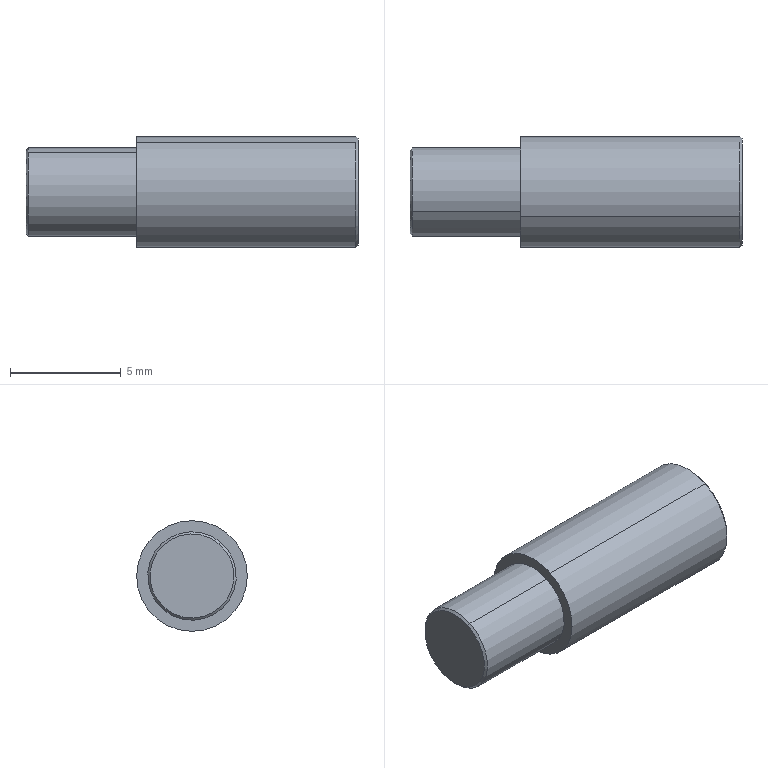Component | SolidWorks | F01AE00111-A2000-21TopEdgeAssembly-1_F01AE00111-A2000-19TopEdgeRollerAssembly-1_F01AE00111-A2008-1 | 1 solid | 11 faces | box 15 x 5 x 5 mm | volume 259 mm3 | cone 4 | cylinder 4 | plane 3 | commonest cylinder face diameters 5 x2 4 x2 | material AISI 304
build123d program:
from build123d import *

# Parameters (mm, degrees)
CHAMFER1_SIZE = 0.1


with BuildPart() as part:
    # Sketch1 → Revolve1 (revolve)
    with BuildSketch(Plane.XY, mode=Mode.PRIVATE) as revolve1_sk:
        Polygon((0, 15), (2, 15), (2, 10), (2.5, 10), (2.5, 0), (0, 0), align=None)
    revolve(revolve1_sk.sketch.rotate(Axis((0, 0, 0), (0, 1, 0)), 90), axis=Axis((0, 0, 0), (0, 1, 0)))

    # Chamfer1
    chamfer1_edges = [part.edges().sort_by_distance(p)[0] for p in [
        (0, 0, 2.5),
        (0, 15, 2),
    ]]
    chamfer(chamfer1_edges, length=CHAMFER1_SIZE)


solid = part.part

# Placed as in the assembly
solid = solid.moved(Location((-133.852, 75.398, -381.975), (0, 0, 90)))
STEP:
#1=COLOUR_RGB('',0.7922,0.8196,0.9333);
#2=FILL_AREA_STYLE_COLOUR('',#1);
#3=FILL_AREA_STYLE('',(#2));
#4=SURFACE_STYLE_FILL_AREA(#3);
#5=SURFACE_SIDE_STYLE('',(#4));
#6=SURFACE_STYLE_USAGE(.BOTH.,#5);
#7=PRESENTATION_STYLE_ASSIGNMENT((#6));
#8=CARTESIAN_POINT('',(-5.86,2.936,-14.971));
#9=VERTEX_POINT('',#8);
#10=CARTESIAN_POINT('',(-5.86,3.001,-15.106));
#11=VERTEX_POINT('',#10);
#12=CARTESIAN_POINT('',(-5.86,2.968,-15.038));
#13=DIRECTION('',(-1.,-0.,-0.));
#14=DIRECTION('',(0.,-0.4399,0.898));
#15=AXIS2_PLACEMENT_3D('',#12,#13,#14);
#16=CIRCLE('',#15,0.0748);
#17=EDGE_CURVE('',#9,#11,#16,.T.);
#18=ORIENTED_EDGE('',*,*,#17,.F.);
#19=CARTESIAN_POINT('',(-5.856,2.934,-14.968));
#20=VERTEX_POINT('',#19);
#21=CARTESIAN_POINT('',(-5.856,2.934,-14.968));
#22=DIRECTION('',(0.7071,-0.3111,0.635));
#23=VECTOR('',#22,39.37);
#24=LINE('',#21,#23);
#25=EDGE_CURVE('',#9,#20,#24,.T.);
#26=ORIENTED_EDGE('',*,*,#25,.T.);
#27=CARTESIAN_POINT('',(-5.856,3.003,-15.109));
#28=VERTEX_POINT('',#27);
#29=CARTESIAN_POINT('',(-5.856,2.968,-15.038));
#30=DIRECTION('',(1.,0.,0.));
#31=DIRECTION('',(0.,-0.4399,0.898));
#32=AXIS2_PLACEMENT_3D('',#29,#30,#31);
#33=CIRCLE('',#32,0.07874);
#34=EDGE_CURVE('',#28,#20,#33,.T.);
#35=ORIENTED_EDGE('',*,*,#34,.F.);
#36=CARTESIAN_POINT('',(-5.856,3.003,-15.109));
#37=DIRECTION('',(0.7071,0.3111,-0.635));
#38=VECTOR('',#37,39.37);
#39=LINE('',#36,#38);
#40=EDGE_CURVE('',#11,#28,#39,.T.);
#41=ORIENTED_EDGE('',*,*,#40,.F.);
#42=EDGE_LOOP('',(#18,#26,#35,#41));
#43=FACE_OUTER_BOUND('',#42,.T.);
#44=CARTESIAN_POINT('',(-5.856,2.968,-15.038));
#45=DIRECTION('',(1.,0.,0.));
#46=DIRECTION('',(0.,0.4399,-0.898));
#47=AXIS2_PLACEMENT_3D('',#44,#45,#46);
#48=CONICAL_SURFACE('',#47,0.07874,0.7854);
#49=ADVANCED_FACE('',(#43),#48,.T.);
#50=CARTESIAN_POINT('',(-5.27,3.01,-15.123));
#51=VERTEX_POINT('',#50);
#52=CARTESIAN_POINT('',(-5.27,2.927,-14.954));
#53=VERTEX_POINT('',#52);
#54=CARTESIAN_POINT('',(-5.27,2.968,-15.038));
#55=DIRECTION('',(1.,0.,0.));
#56=DIRECTION('',(0.,0.4399,-0.898));
#57=AXIS2_PLACEMENT_3D('',#54,#55,#56);
#58=CIRCLE('',#57,0.09449);
#59=EDGE_CURVE('',#51,#53,#58,.T.);
#60=ORIENTED_EDGE('',*,*,#59,.F.);
#61=CARTESIAN_POINT('',(-5.274,3.012,-15.127));
#62=VERTEX_POINT('',#61);
#63=CARTESIAN_POINT('',(-5.27,3.01,-15.123));
#64=DIRECTION('',(-0.7071,0.3111,-0.635));
#65=VECTOR('',#64,39.37);
#66=LINE('',#63,#65);
#67=EDGE_CURVE('',#51,#62,#66,.T.);
#68=ORIENTED_EDGE('',*,*,#67,.T.);
#69=CARTESIAN_POINT('',(-5.274,2.925,-14.95));
#70=VERTEX_POINT('',#69);
#71=CARTESIAN_POINT('',(-5.274,2.968,-15.038));
#72=DIRECTION('',(-1.,-0.,-0.));
#73=DIRECTION('',(0.,0.4399,-0.898));
#74=AXIS2_PLACEMENT_3D('',#71,#72,#73);
#75=CIRCLE('',#74,0.09843);
#76=EDGE_CURVE('',#70,#62,#75,.T.);
#77=ORIENTED_EDGE('',*,*,#76,.F.);
#78=CARTESIAN_POINT('',(-5.27,2.927,-14.954));
#79=DIRECTION('',(-0.7071,-0.3111,0.635));
#80=VECTOR('',#79,39.37);
#81=LINE('',#78,#80);
#82=EDGE_CURVE('',#53,#70,#81,.T.);
#83=ORIENTED_EDGE('',*,*,#82,.F.);
#84=EDGE_LOOP('',(#60,#68,#77,#83));
#85=FACE_OUTER_BOUND('',#84,.T.);
#86=CARTESIAN_POINT('',(-5.27,2.968,-15.038));
#87=DIRECTION('',(-1.,-0.,-0.));
#88=DIRECTION('',(0.,-0.4399,0.898));
#89=AXIS2_PLACEMENT_3D('',#86,#87,#88);
#90=CONICAL_SURFACE('',#89,0.09449,0.7854);
#91=ADVANCED_FACE('',(#85),#90,.T.);
#92=CARTESIAN_POINT('',(-5.663,3.012,-15.127));
#93=VERTEX_POINT('',#92);
#94=CARTESIAN_POINT('',(-5.663,2.925,-14.95));
#95=VERTEX_POINT('',#94);
#96=CARTESIAN_POINT('',(-5.663,2.968,-15.038));
#97=DIRECTION('',(1.,0.,0.));
#98=DIRECTION('',(0.,0.4399,-0.898));
#99=AXIS2_PLACEMENT_3D('',#96,#97,#98);
#100=CIRCLE('',#99,0.09843);
#101=EDGE_CURVE('',#93,#95,#100,.T.);
#102=ORIENTED_EDGE('',*,*,#101,.T.);
#103=CARTESIAN_POINT('',(-5.27,2.925,-14.95));
#104=DIRECTION('',(1.,0.,0.));
#105=VECTOR('',#104,39.37);
#106=LINE('',#103,#105);
#107=EDGE_CURVE('',#95,#70,#106,.T.);
#108=ORIENTED_EDGE('',*,*,#107,.T.);
#109=ORIENTED_EDGE('',*,*,#76,.T.);
#110=CARTESIAN_POINT('',(-5.27,3.012,-15.127));
#111=DIRECTION('',(1.,0.,0.));
#112=VECTOR('',#111,39.37);
#113=LINE('',#110,#112);
#114=EDGE_CURVE('',#93,#62,#113,.T.);
#115=ORIENTED_EDGE('',*,*,#114,.F.);
#116=EDGE_LOOP('',(#102,#108,#109,#115));
#117=FACE_OUTER_BOUND('',#116,.T.);
#118=CARTESIAN_POINT('',(-5.27,2.968,-15.038));
#119=DIRECTION('',(1.,0.,0.));
#120=DIRECTION('',(0.,0.4399,-0.898));
#121=AXIS2_PLACEMENT_3D('',#118,#119,#120);
#122=CYLINDRICAL_SURFACE('',#121,0.09843);
#123=ADVANCED_FACE('',(#117),#122,.T.);
#124=ORIENTED_EDGE('',*,*,#34,.T.);
#125=CARTESIAN_POINT('',(-5.663,2.934,-14.968));
#126=VERTEX_POINT('',#125);
#127=CARTESIAN_POINT('',(-5.27,2.934,-14.968));
#128=DIRECTION('',(1.,0.,0.));
#129=VECTOR('',#128,39.37);
#130=LINE('',#127,#129);
#131=EDGE_CURVE('',#20,#126,#130,.T.);
#132=ORIENTED_EDGE('',*,*,#131,.T.);
#133=CARTESIAN_POINT('',(-5.663,3.003,-15.109));
#134=VERTEX_POINT('',#133);
#135=CARTESIAN_POINT('',(-5.663,2.968,-15.038));
#136=DIRECTION('',(1.,0.,0.));
#137=DIRECTION('',(0.,0.4399,-0.898));
#138=AXIS2_PLACEMENT_3D('',#135,#136,#137);
#139=CIRCLE('',#138,0.07874);
#140=EDGE_CURVE('',#134,#126,#139,.T.);
#141=ORIENTED_EDGE('',*,*,#140,.F.);
#142=CARTESIAN_POINT('',(-5.27,3.003,-15.109));
#143=DIRECTION('',(1.,0.,0.));
#144=VECTOR('',#143,39.37);
#145=LINE('',#142,#144);
#146=EDGE_CURVE('',#28,#134,#145,.T.);
#147=ORIENTED_EDGE('',*,*,#146,.F.);
#148=EDGE_LOOP('',(#124,#132,#141,#147));
#149=FACE_OUTER_BOUND('',#148,.T.);
#150=CARTESIAN_POINT('',(-5.27,2.968,-15.038));
#151=DIRECTION('',(1.,0.,0.));
#152=DIRECTION('',(0.,0.4399,-0.898));
#153=AXIS2_PLACEMENT_3D('',#150,#151,#152);
#154=CYLINDRICAL_SURFACE('',#153,0.07874);
#155=ADVANCED_FACE('',(#149),#154,.T.);
#156=CARTESIAN_POINT('',(-5.86,2.968,-15.038));
#157=DIRECTION('',(-1.,-0.,-0.));
#158=DIRECTION('',(0.,-0.4399,0.898));
#159=AXIS2_PLACEMENT_3D('',#156,#157,#158);
#160=CIRCLE('',#159,0.0748);
#161=EDGE_CURVE('',#11,#9,#160,.T.);
#162=ORIENTED_EDGE('',*,*,#161,.T.);
#163=ORIENTED_EDGE('',*,*,#17,.T.);
#164=EDGE_LOOP('',(#162,#163));
#165=FACE_OUTER_BOUND('',#164,.T.);
#166=CARTESIAN_POINT('',(-5.86,2.968,-15.038));
#167=DIRECTION('',(-1.,-0.,-0.));
#168=DIRECTION('',(-0.,-0.4399,0.898));
#169=AXIS2_PLACEMENT_3D('',#166,#167,#168);
#170=PLANE('',#169);
#171=ADVANCED_FACE('',(#165),#170,.T.);
#172=ORIENTED_EDGE('',*,*,#131,.F.);
#173=CARTESIAN_POINT('',(-5.856,2.968,-15.038));
#174=DIRECTION('',(1.,0.,0.));
#175=DIRECTION('',(0.,-0.4399,0.898));
#176=AXIS2_PLACEMENT_3D('',#173,#174,#175);
#177=CIRCLE('',#176,0.07874);
#178=EDGE_CURVE('',#20,#28,#177,.T.);
#179=ORIENTED_EDGE('',*,*,#178,.T.);
#180=ORIENTED_EDGE('',*,*,#146,.T.);
#181=CARTESIAN_POINT('',(-5.663,2.968,-15.038));
#182=DIRECTION('',(1.,0.,0.));
#183=DIRECTION('',(0.,0.4399,-0.898));
#184=AXIS2_PLACEMENT_3D('',#181,#182,#183);
#185=CIRCLE('',#184,0.07874);
#186=EDGE_CURVE('',#126,#134,#185,.T.);
#187=ORIENTED_EDGE('',*,*,#186,.F.);
#188=EDGE_LOOP('',(#172,#179,#180,#187));
#189=FACE_OUTER_BOUND('',#188,.T.);
#190=CARTESIAN_POINT('',(-5.27,2.968,-15.038));
#191=DIRECTION('',(1.,0.,0.));
#192=DIRECTION('',(0.,0.4399,-0.898));
#193=AXIS2_PLACEMENT_3D('',#190,#191,#192);
#194=CYLINDRICAL_SURFACE('',#193,0.07874);
#195=ADVANCED_FACE('',(#189),#194,.T.);
#196=ORIENTED_EDGE('',*,*,#140,.T.);
#197=ORIENTED_EDGE('',*,*,#186,.T.);
#198=EDGE_LOOP('',(#196,#197));
#199=FACE_BOUND('',#198,.T.);
#200=ORIENTED_EDGE('',*,*,#101,.F.);
#201=CARTESIAN_POINT('',(-5.663,2.968,-15.038));
#202=DIRECTION('',(1.,0.,0.));
#203=DIRECTION('',(0.,0.4399,-0.898));
#204=AXIS2_PLACEMENT_3D('',#201,#202,#203);
#205=CIRCLE('',#204,0.09843);
#206=EDGE_CURVE('',#95,#93,#205,.T.);
#207=ORIENTED_EDGE('',*,*,#206,.F.);
#208=EDGE_LOOP('',(#200,#207));
#209=FACE_OUTER_BOUND('',#208,.T.);
#210=CARTESIAN_POINT('',(-5.663,3.039,-15.004));
#211=DIRECTION('',(-1.,-0.,-0.));
#212=DIRECTION('',(-0.,-0.4399,0.898));
#213=AXIS2_PLACEMENT_3D('',#210,#211,#212);
#214=PLANE('',#213);
#215=ADVANCED_FACE('',(#199,#209),#214,.T.);
#216=ORIENTED_EDGE('',*,*,#107,.F.);
#217=ORIENTED_EDGE('',*,*,#206,.T.);
#218=ORIENTED_EDGE('',*,*,#114,.T.);
#219=CARTESIAN_POINT('',(-5.274,2.968,-15.038));
#220=DIRECTION('',(-1.,-0.,-0.));
#221=DIRECTION('',(0.,0.4399,-0.898));
#222=AXIS2_PLACEMENT_3D('',#219,#220,#221);
#223=CIRCLE('',#222,0.09843);
#224=EDGE_CURVE('',#62,#70,#223,.T.);
#225=ORIENTED_EDGE('',*,*,#224,.T.);
#226=EDGE_LOOP('',(#216,#217,#218,#225));
#227=FACE_OUTER_BOUND('',#226,.T.);
#228=CARTESIAN_POINT('',(-5.27,2.968,-15.038));
#229=DIRECTION('',(1.,0.,0.));
#230=DIRECTION('',(0.,0.4399,-0.898));
#231=AXIS2_PLACEMENT_3D('',#228,#229,#230);
#232=CYLINDRICAL_SURFACE('',#231,0.09843);
#233=ADVANCED_FACE('',(#227),#232,.T.);
#234=CARTESIAN_POINT('',(-5.27,2.968,-15.038));
#235=DIRECTION('',(1.,0.,0.));
#236=DIRECTION('',(0.,0.4399,-0.898));
#237=AXIS2_PLACEMENT_3D('',#234,#235,#236);
#238=CIRCLE('',#237,0.09449);
#239=EDGE_CURVE('',#53,#51,#238,.T.);
#240=ORIENTED_EDGE('',*,*,#239,.T.);
#241=ORIENTED_EDGE('',*,*,#59,.T.);
#242=EDGE_LOOP('',(#240,#241));
#243=FACE_OUTER_BOUND('',#242,.T.);
#244=CARTESIAN_POINT('',(-5.27,3.057,-14.995));
#245=DIRECTION('',(1.,0.,0.));
#246=DIRECTION('',(0.,0.4399,-0.898));
#247=AXIS2_PLACEMENT_3D('',#244,#245,#246);
#248=PLANE('',#247);
#249=ADVANCED_FACE('',(#243),#248,.T.);
#250=ORIENTED_EDGE('',*,*,#67,.F.);
#251=ORIENTED_EDGE('',*,*,#239,.F.);
#252=ORIENTED_EDGE('',*,*,#82,.T.);
#253=ORIENTED_EDGE('',*,*,#224,.F.);
#254=EDGE_LOOP('',(#250,#251,#252,#253));
#255=FACE_OUTER_BOUND('',#254,.T.);
#256=CARTESIAN_POINT('',(-5.27,2.968,-15.038));
#257=DIRECTION('',(-1.,-0.,-0.));
#258=DIRECTION('',(0.,-0.4399,0.898));
#259=AXIS2_PLACEMENT_3D('',#256,#257,#258);
#260=CONICAL_SURFACE('',#259,0.09449,0.7854);
#261=ADVANCED_FACE('',(#255),#260,.T.);
#262=ORIENTED_EDGE('',*,*,#25,.F.);
#263=ORIENTED_EDGE('',*,*,#161,.F.);
#264=ORIENTED_EDGE('',*,*,#40,.T.);
#265=ORIENTED_EDGE('',*,*,#178,.F.);
#266=EDGE_LOOP('',(#262,#263,#264,#265));
#267=FACE_OUTER_BOUND('',#266,.T.);
#268=CARTESIAN_POINT('',(-5.856,2.968,-15.038));
#269=DIRECTION('',(1.,0.,0.));
#270=DIRECTION('',(0.,0.4399,-0.898));
#271=AXIS2_PLACEMENT_3D('',#268,#269,#270);
#272=CONICAL_SURFACE('',#271,0.07874,0.7854);
#273=ADVANCED_FACE('',(#267),#272,.T.);
#274=CLOSED_SHELL('',(#49,#91,#123,#155,#171,#195,#215,#233,#249,#261,#273));
#275=MANIFOLD_SOLID_BREP('',#274);
#276=STYLED_ITEM('',(#7),#275);
#277=(LENGTH_UNIT()NAMED_UNIT(*)SI_UNIT($,.METRE.));
#278=LENGTH_MEASURE_WITH_UNIT(LENGTH_MEASURE(0.0254),#277);
#279=DIMENSIONAL_EXPONENTS(1.,0.,0.,0.,0.,0.,0.);
#280=(CONVERSION_BASED_UNIT('',#278)LENGTH_UNIT()NAMED_UNIT(#279));
#281=UNCERTAINTY_MEASURE_WITH_UNIT(LENGTH_MEASURE(0.00001),#280,'','');
#282=(NAMED_UNIT(*)PLANE_ANGLE_UNIT()SI_UNIT($,.RADIAN.));
#283=(NAMED_UNIT(*)SI_UNIT($,.STERADIAN.)SOLID_ANGLE_UNIT());
#284=(GEOMETRIC_REPRESENTATION_CONTEXT(3)GLOBAL_UNCERTAINTY_ASSIGNED_CONTEXT((#281))GLOBAL_UNIT_ASSIGNED_CONTEXT((#280,#282,#283))REPRESENTATION_CONTEXT('',''));
#285=MECHANICAL_DESIGN_GEOMETRIC_PRESENTATION_REPRESENTATION('',(#276),#284);
#286=CARTESIAN_POINT('',(0.,0.,0.));
#287=DIRECTION('',(0.,0.,1.));
#288=DIRECTION('',(1.,0.,0.));
#289=AXIS2_PLACEMENT_3D('',#286,#287,#288);
#290=(LENGTH_UNIT()NAMED_UNIT(*)SI_UNIT($,.METRE.));
#291=LENGTH_MEASURE_WITH_UNIT(LENGTH_MEASURE(0.0254),#290);
#292=DIMENSIONAL_EXPONENTS(1.,0.,0.,0.,0.,0.,0.);
#293=(CONVERSION_BASED_UNIT('',#291)LENGTH_UNIT()NAMED_UNIT(#292));
#294=UNCERTAINTY_MEASURE_WITH_UNIT(LENGTH_MEASURE(0.00001),#293,'','');
#295=(NAMED_UNIT(*)PLANE_ANGLE_UNIT()SI_UNIT($,.RADIAN.));
#296=(NAMED_UNIT(*)SI_UNIT($,.STERADIAN.)SOLID_ANGLE_UNIT());
#297=(GEOMETRIC_REPRESENTATION_CONTEXT(3)GLOBAL_UNCERTAINTY_ASSIGNED_CONTEXT((#294))GLOBAL_UNIT_ASSIGNED_CONTEXT((#293,#295,#296))REPRESENTATION_CONTEXT('',''));
#298=ADVANCED_BREP_SHAPE_REPRESENTATION('',(#275,#289),#297);
#299=PRESENTATION_LAYER_ASSIGNMENT('','',(#276));